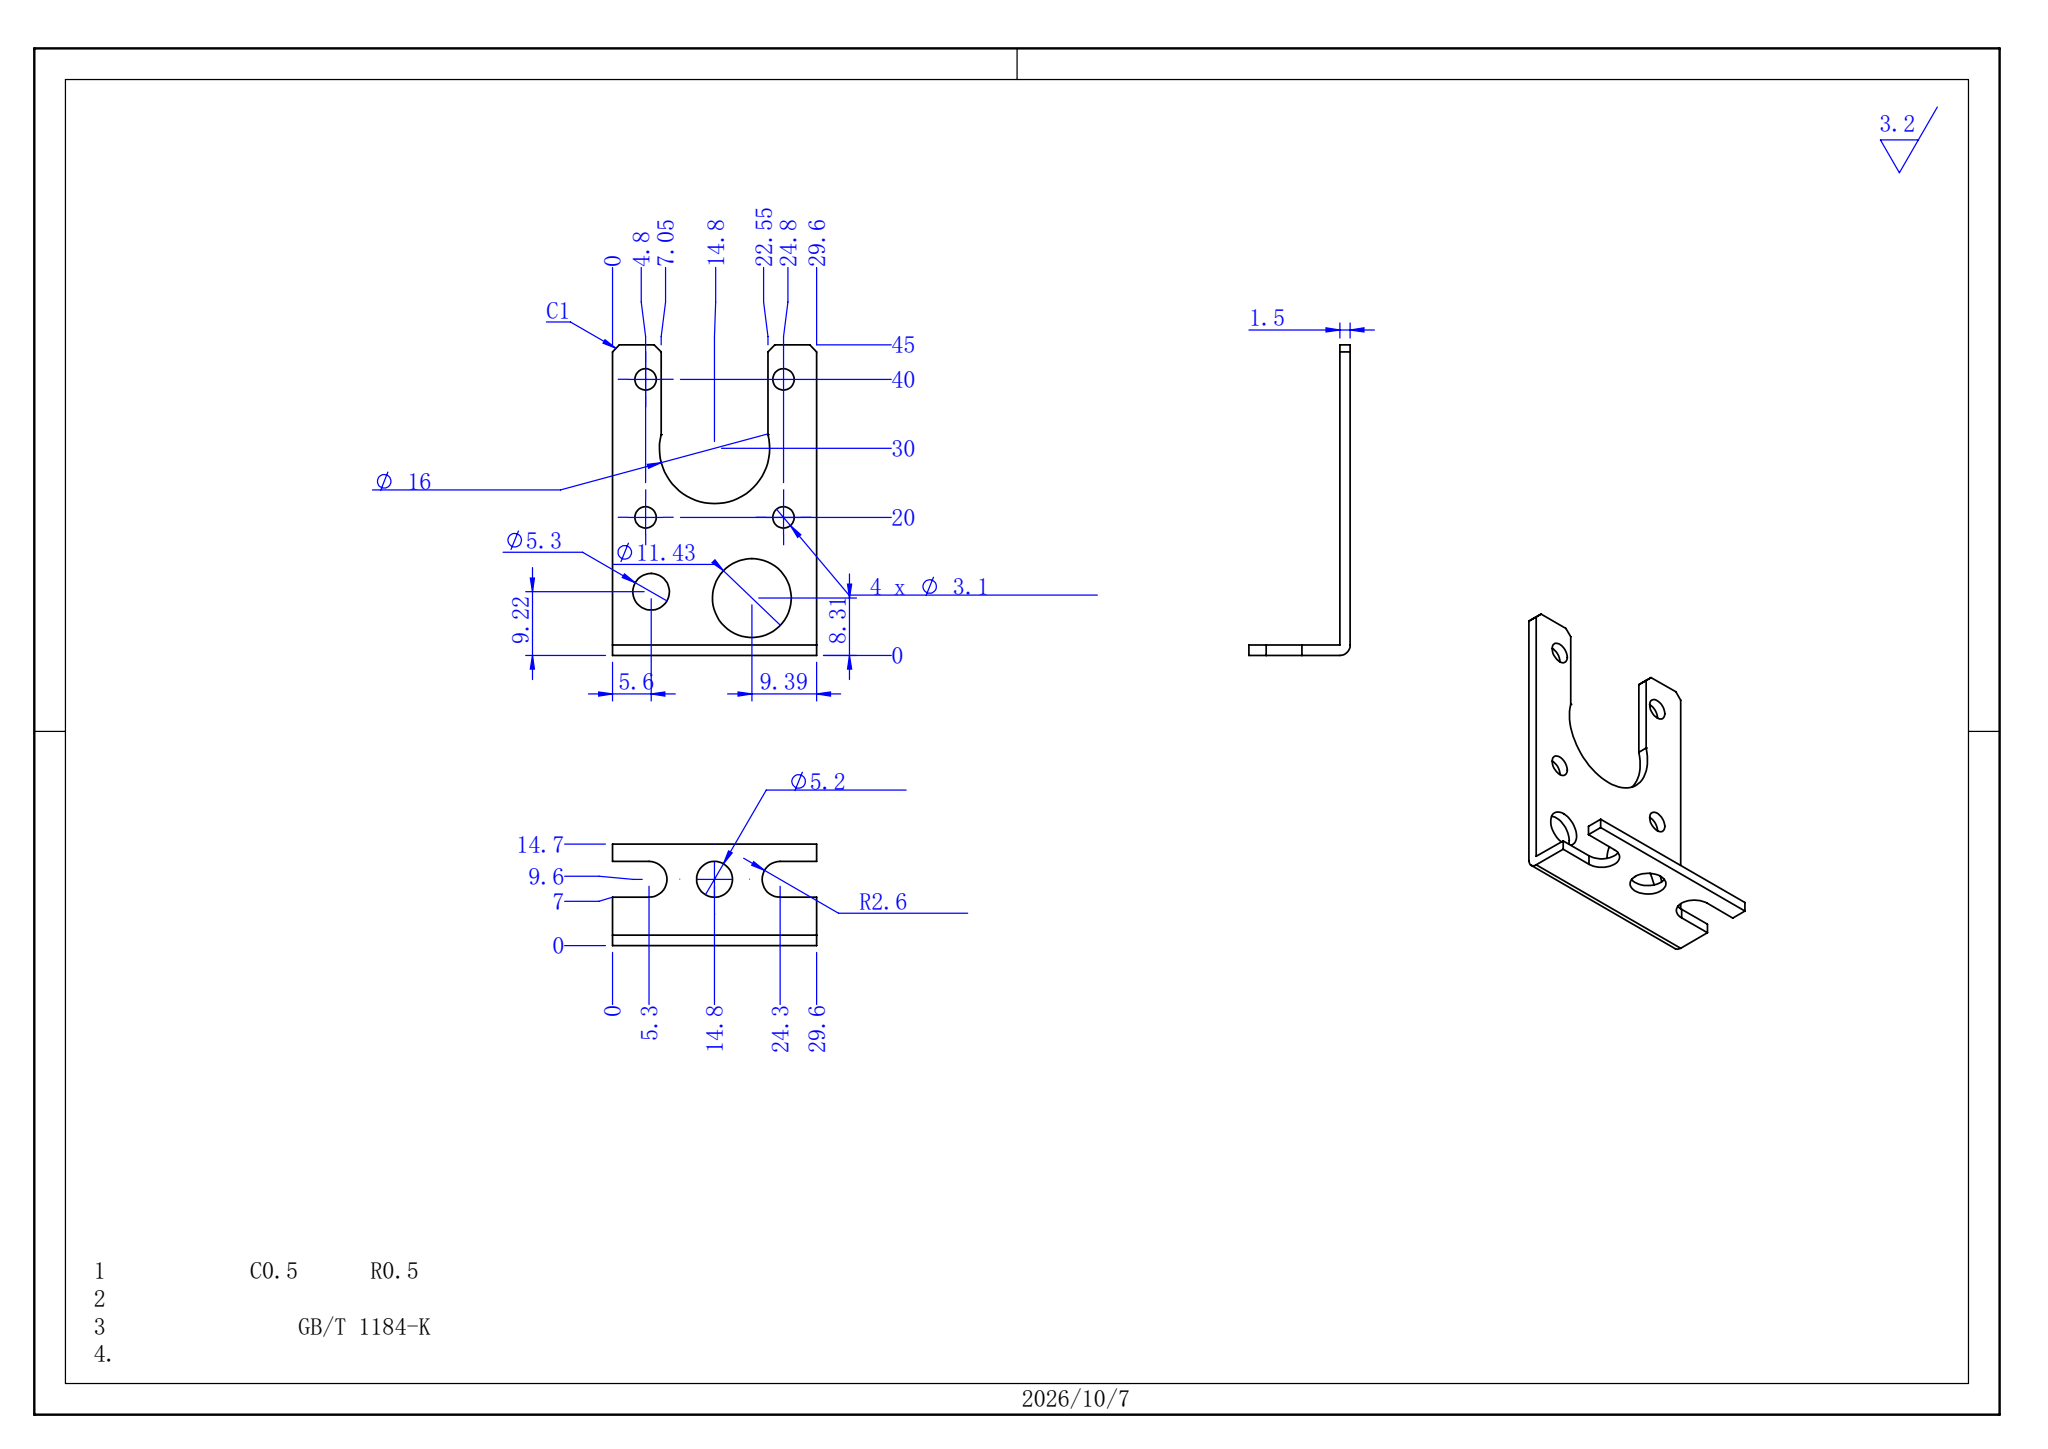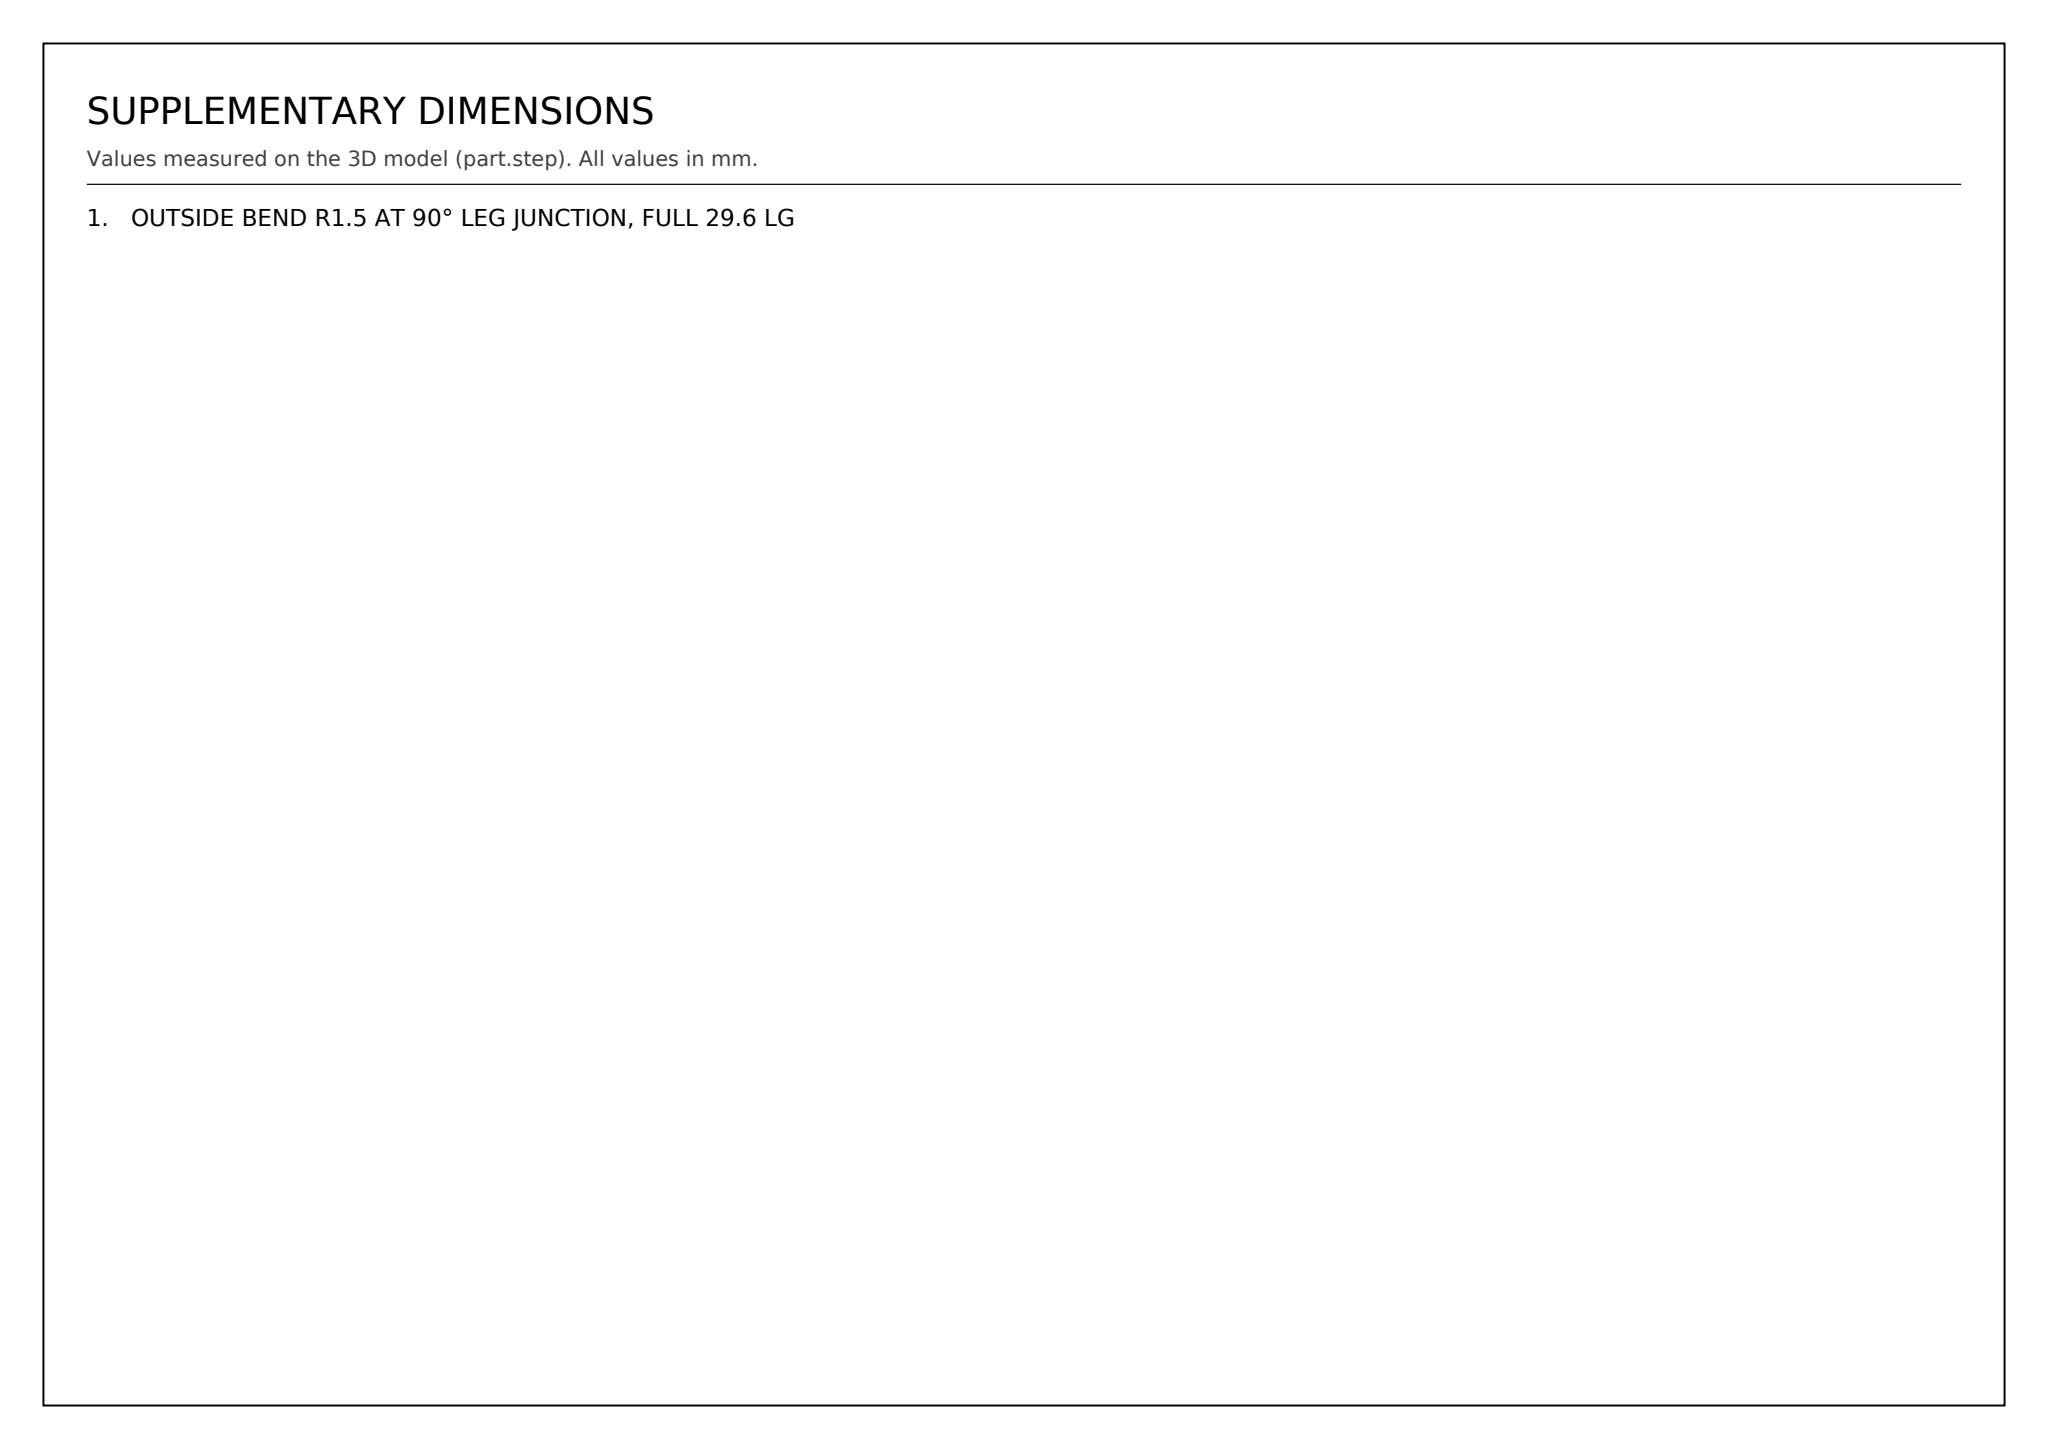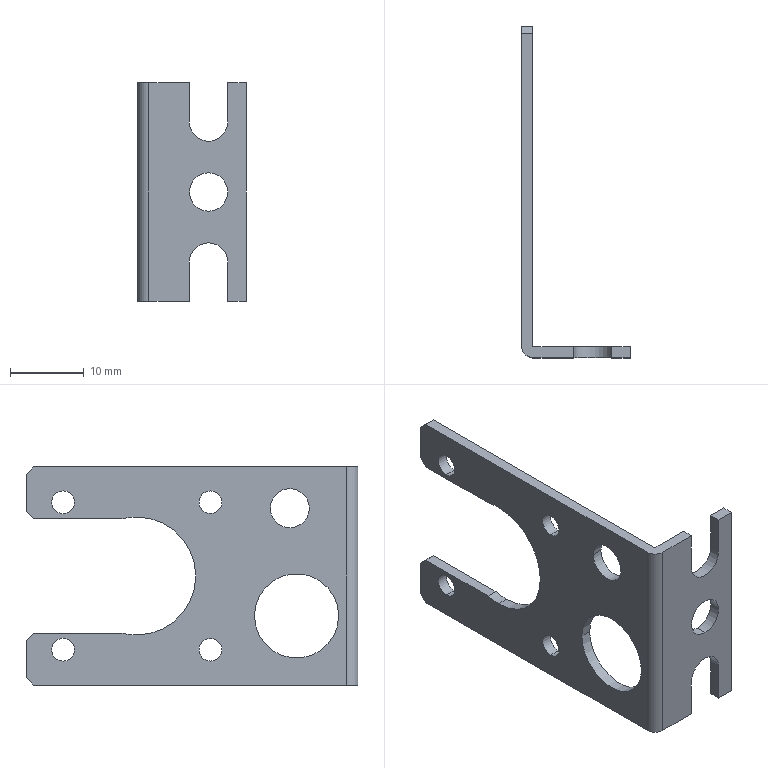Part | SolidWorks | mm | 1 solid | 44 faces | box 14.7 x 45 x 29.6 mm | volume 1688 mm3 | plane 23 | cylinder 21 | commonest cylinder face diameters 3.1 x8 5.2 x5 16 x3 5.305 x2 11.427 x2 3 x1
Drawing notes:
OUTSIDE BEND R1.5 AT 90° LEG JUNCTION, FULL 29.6 LG | from the solid: cylinder dia 3.0 axis z at (x=1.5,y=1.5), length 29.6; tangent to outer faces x=0 and y=0 (planes x=0,y=0; inner faces x=1.5,y=1.5 thk 1.5)
build123d program:
from build123d import *

# Parameters (mm, degrees)
BOSS_EXTRUDE1_DEPTH        = 29.6
FILLET1_R                  = 1.5
SKETCH2_R                  = 2.6
CUT_EXTRUDE1_DEPTH         = 55.631
F_3_1_3_1_DIAMETER_HOLE1_D = 3.1
F_16_0_16_DIAMETER_HOLE1_D = 16
SKETCH7_W                  = 15.5
SKETCH7_H                  = 13
CUT_EXTRUDE2_DEPTH         = 56.832
CHAMFER3_SIZE              = 1
SKETCH8_R                  = 2.652
SKETCH8_R_2                = 5.713
CUT_EXTRUDE3_DEPTH         = 10


with BuildPart() as part:
    # Sketch1 → Boss-Extrude1 (new body)
    with BuildSketch(Plane.XY):
        Polygon((1.5, 45), (1.5, 1.5), (14.7, 1.5), (14.7, 0), (0, 0), (0, 45), align=None)
    extrude(amount=BOSS_EXTRUDE1_DEPTH)

    # Fillet1
    fillet1_edges = [part.edges().sort_by_distance(p)[0] for p in [
        (0, 0, 14.8),
    ]]
    fillet(fillet1_edges, radius=FILLET1_R)

    # Sketch2 → Cut-Extrude1 (cut, through all)
    with BuildSketch(Plane(origin=(0, 1.5, 0), x_dir=(1, 0, 0), z_dir=(0, 1, 0))):
        with Locations(Location((9.6, -14.8, 0), (0, 0, 270))):
            Circle(SKETCH2_R)
        with BuildLine():
            Line((7, -5.3), (7, 0))
            Line((7, 0), (12.2, 0))
            Line((12.2, 0), (12.2, -5.3))
            ThreePointArc((12.2, -5.3), (9.6, -7.9), (7, -5.3))
        make_face()
        with BuildLine():
            Line((7, -24.3), (7, -29.6))
            Line((7, -29.6), (12.2, -29.6))
            Line((12.2, -29.6), (12.2, -24.3))
            ThreePointArc((12.2, -24.3), (9.6, -21.7), (7, -24.3))
        make_face()
    extrude(amount=-CUT_EXTRUDE1_DEPTH, mode=Mode.SUBTRACT)

    # 3.1 _3.1_ Diameter Hole1 (through all)
    with Locations(Plane(origin=(1.5, 0, 0), x_dir=(0, 0, -1), z_dir=(1, 0, 0))):
        with Locations((-4.8, 40), (-24.8, 40), (-24.8, 20), (-4.8, 20)):
            Hole(F_3_1_3_1_DIAMETER_HOLE1_D / 2)

    # 16.0 _16_ Diameter Hole1 (through all)
    with Locations(Plane(origin=(1.5, 0, 0), x_dir=(0, 0, -1), z_dir=(1, 0, 0))):
        with Locations((-14.8, 30)):
            Hole(F_16_0_16_DIAMETER_HOLE1_D / 2)

    # Sketch7 → Cut-Extrude2 (cut, through all)
    with BuildSketch(Plane.ZY):
        with Locations((14.8, 38.5)):
            Rectangle(SKETCH7_W, SKETCH7_H)
    extrude(amount=-CUT_EXTRUDE2_DEPTH, mode=Mode.SUBTRACT)

    # Chamfer3
    chamfer3_edges = [part.edges().sort_by_distance(p)[0] for p in [
        (0.75, 45, 29.6),
        (0.75, 45, 0),
        (0.75, 45, 7.05),
        (0.75, 45, 22.55),
    ]]
    chamfer(chamfer3_edges, length=CHAMFER3_SIZE)

    # Sketch8 → Cut-Extrude3 (cut)
    with BuildSketch(Plane(origin=(1.5, 0, 0), x_dir=(0, 0, -1), z_dir=(1, 0, 0))):
        with Locations(Location((-23.997, 9.223, 0), (0, 0, 90))):
            Circle(SKETCH8_R)
        with Locations(Location((-9.389, 8.314, 0), (0, 0, 90))):
            Circle(SKETCH8_R_2)
    extrude(amount=-CUT_EXTRUDE3_DEPTH, mode=Mode.SUBTRACT)


solid = part.part